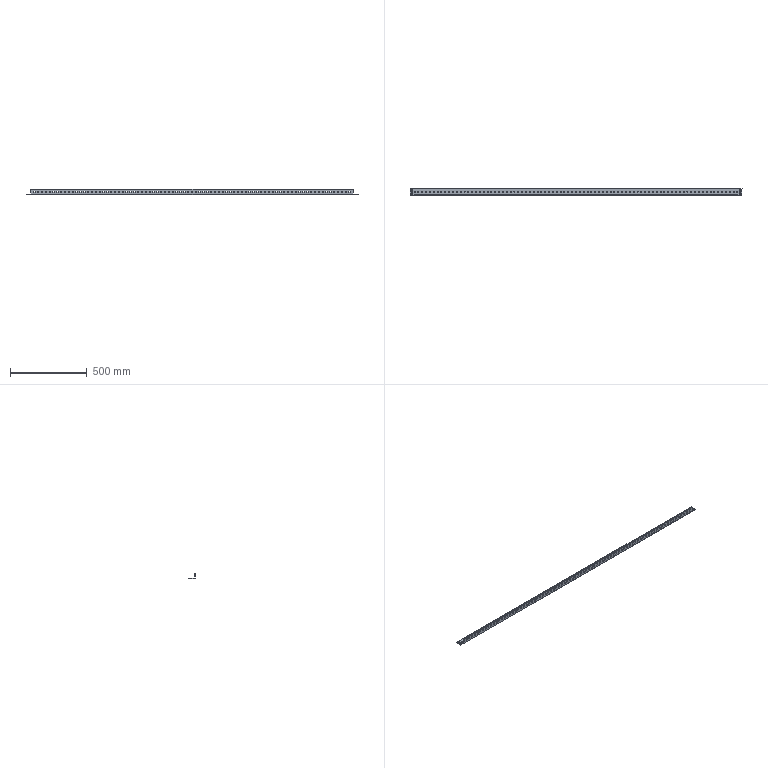Component | SolidWorks | PanelSupportAngleSteelPG50-151-1 | 1 solid | 536 faces | volume 347941 mm3 | plane 352 | cylinder 184 | commonest cylinder face diameters 6.5 x170 6 x12 5.2 x1 0.2 x1